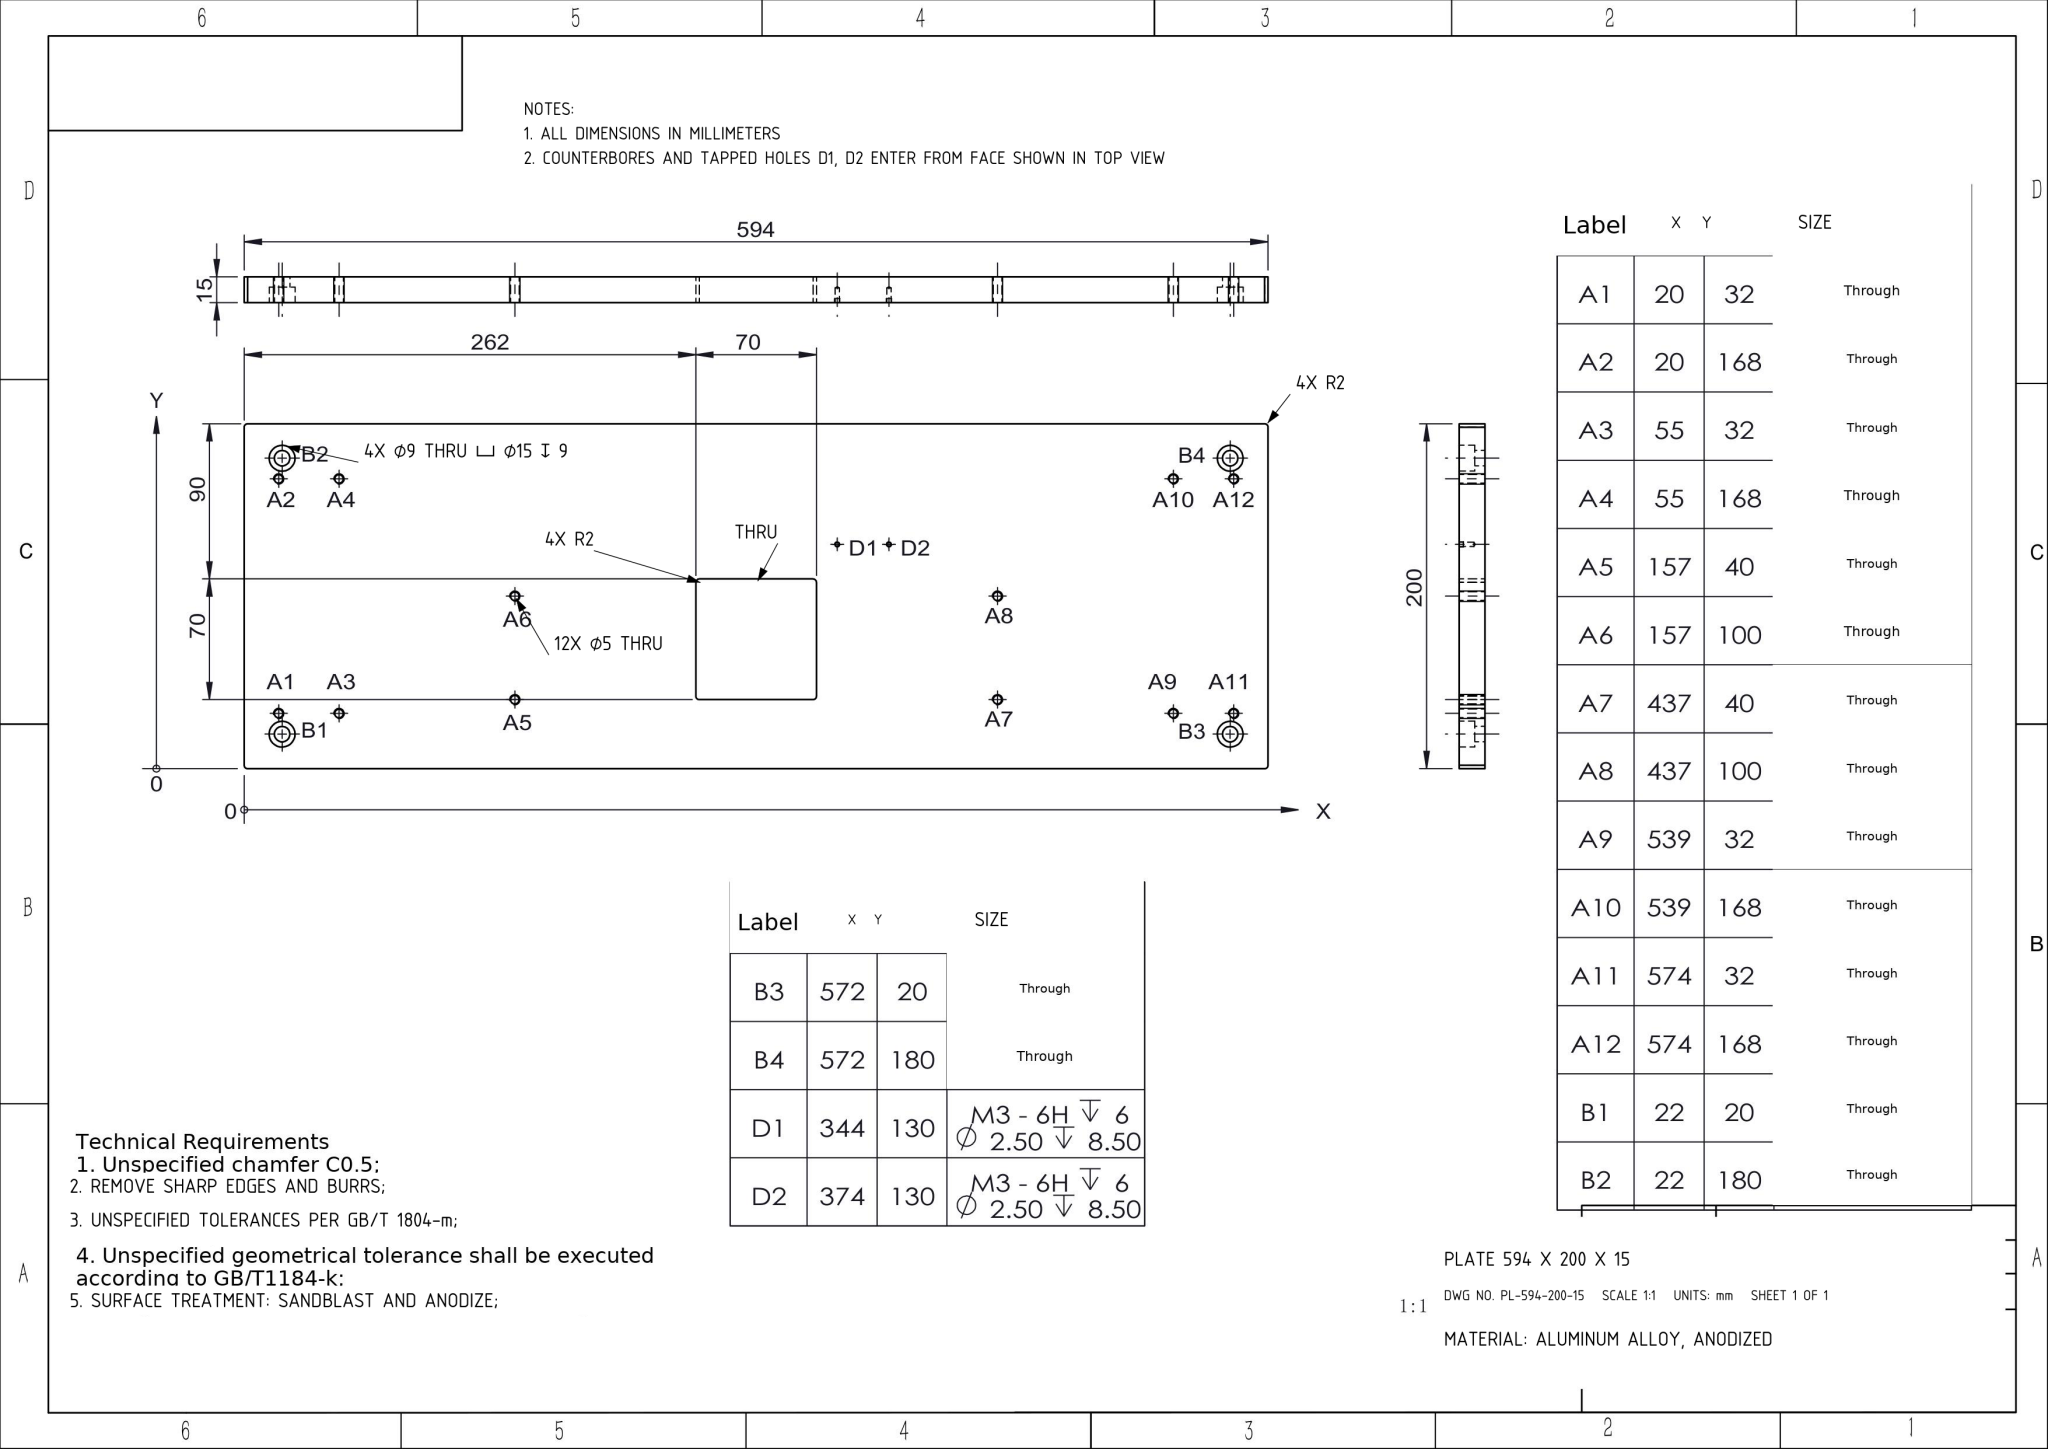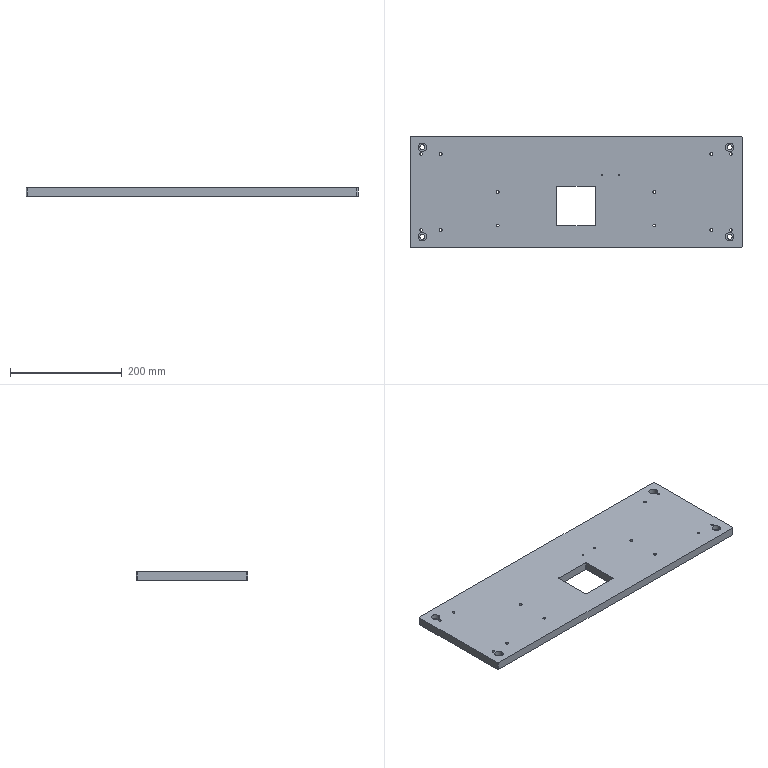Part | NX | mm | 1 solid | 70 faces | box 594 x 200 x 15 mm | volume 1696991 mm3 | cylinder 52 | plane 14 | cone 4 | commonest cylinder face diameters 5 x24 15 x8 9 x8 4 x8 2.5 x4